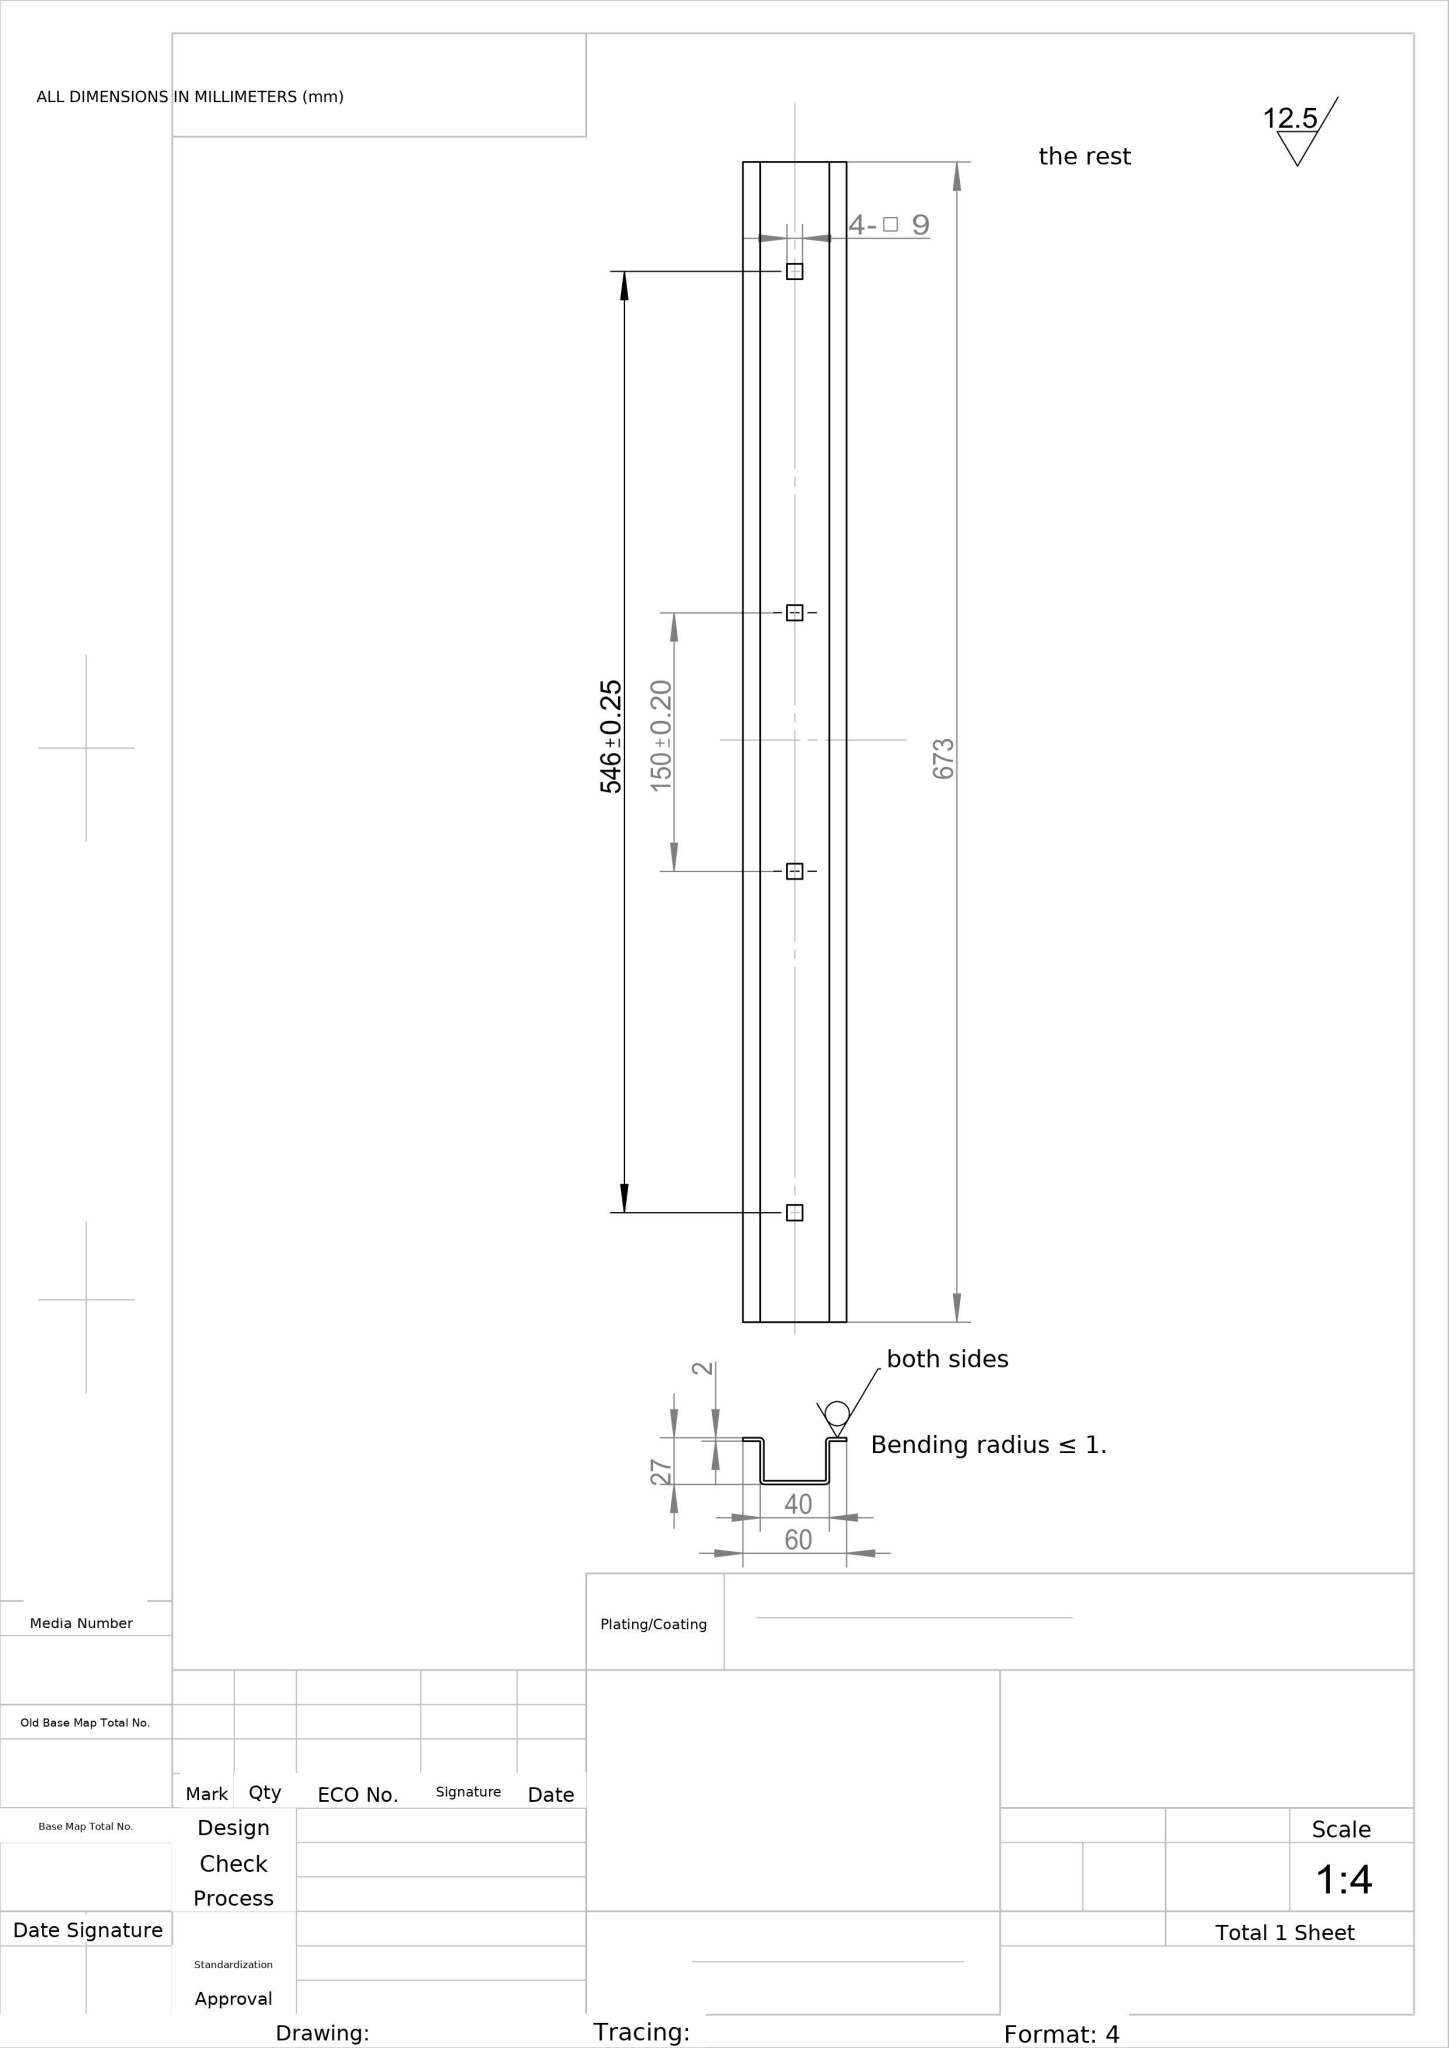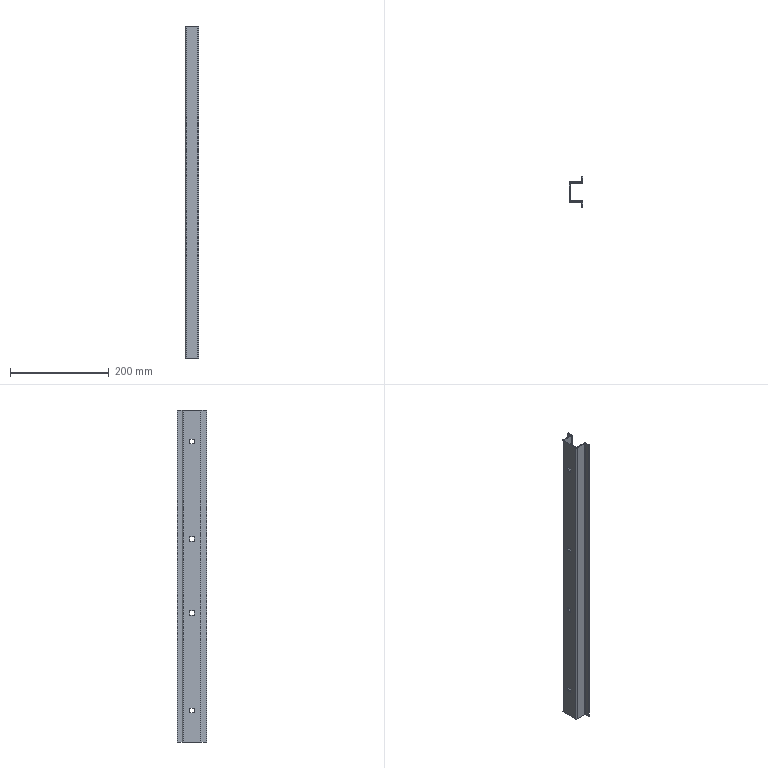Part | NX | mm | 1 solid | 54 faces | box 27 x 60 x 673 mm | volume 144639 mm3 | plane 46 | cylinder 8 | commonest cylinder face diameters 0.4 x4 4.4 x4